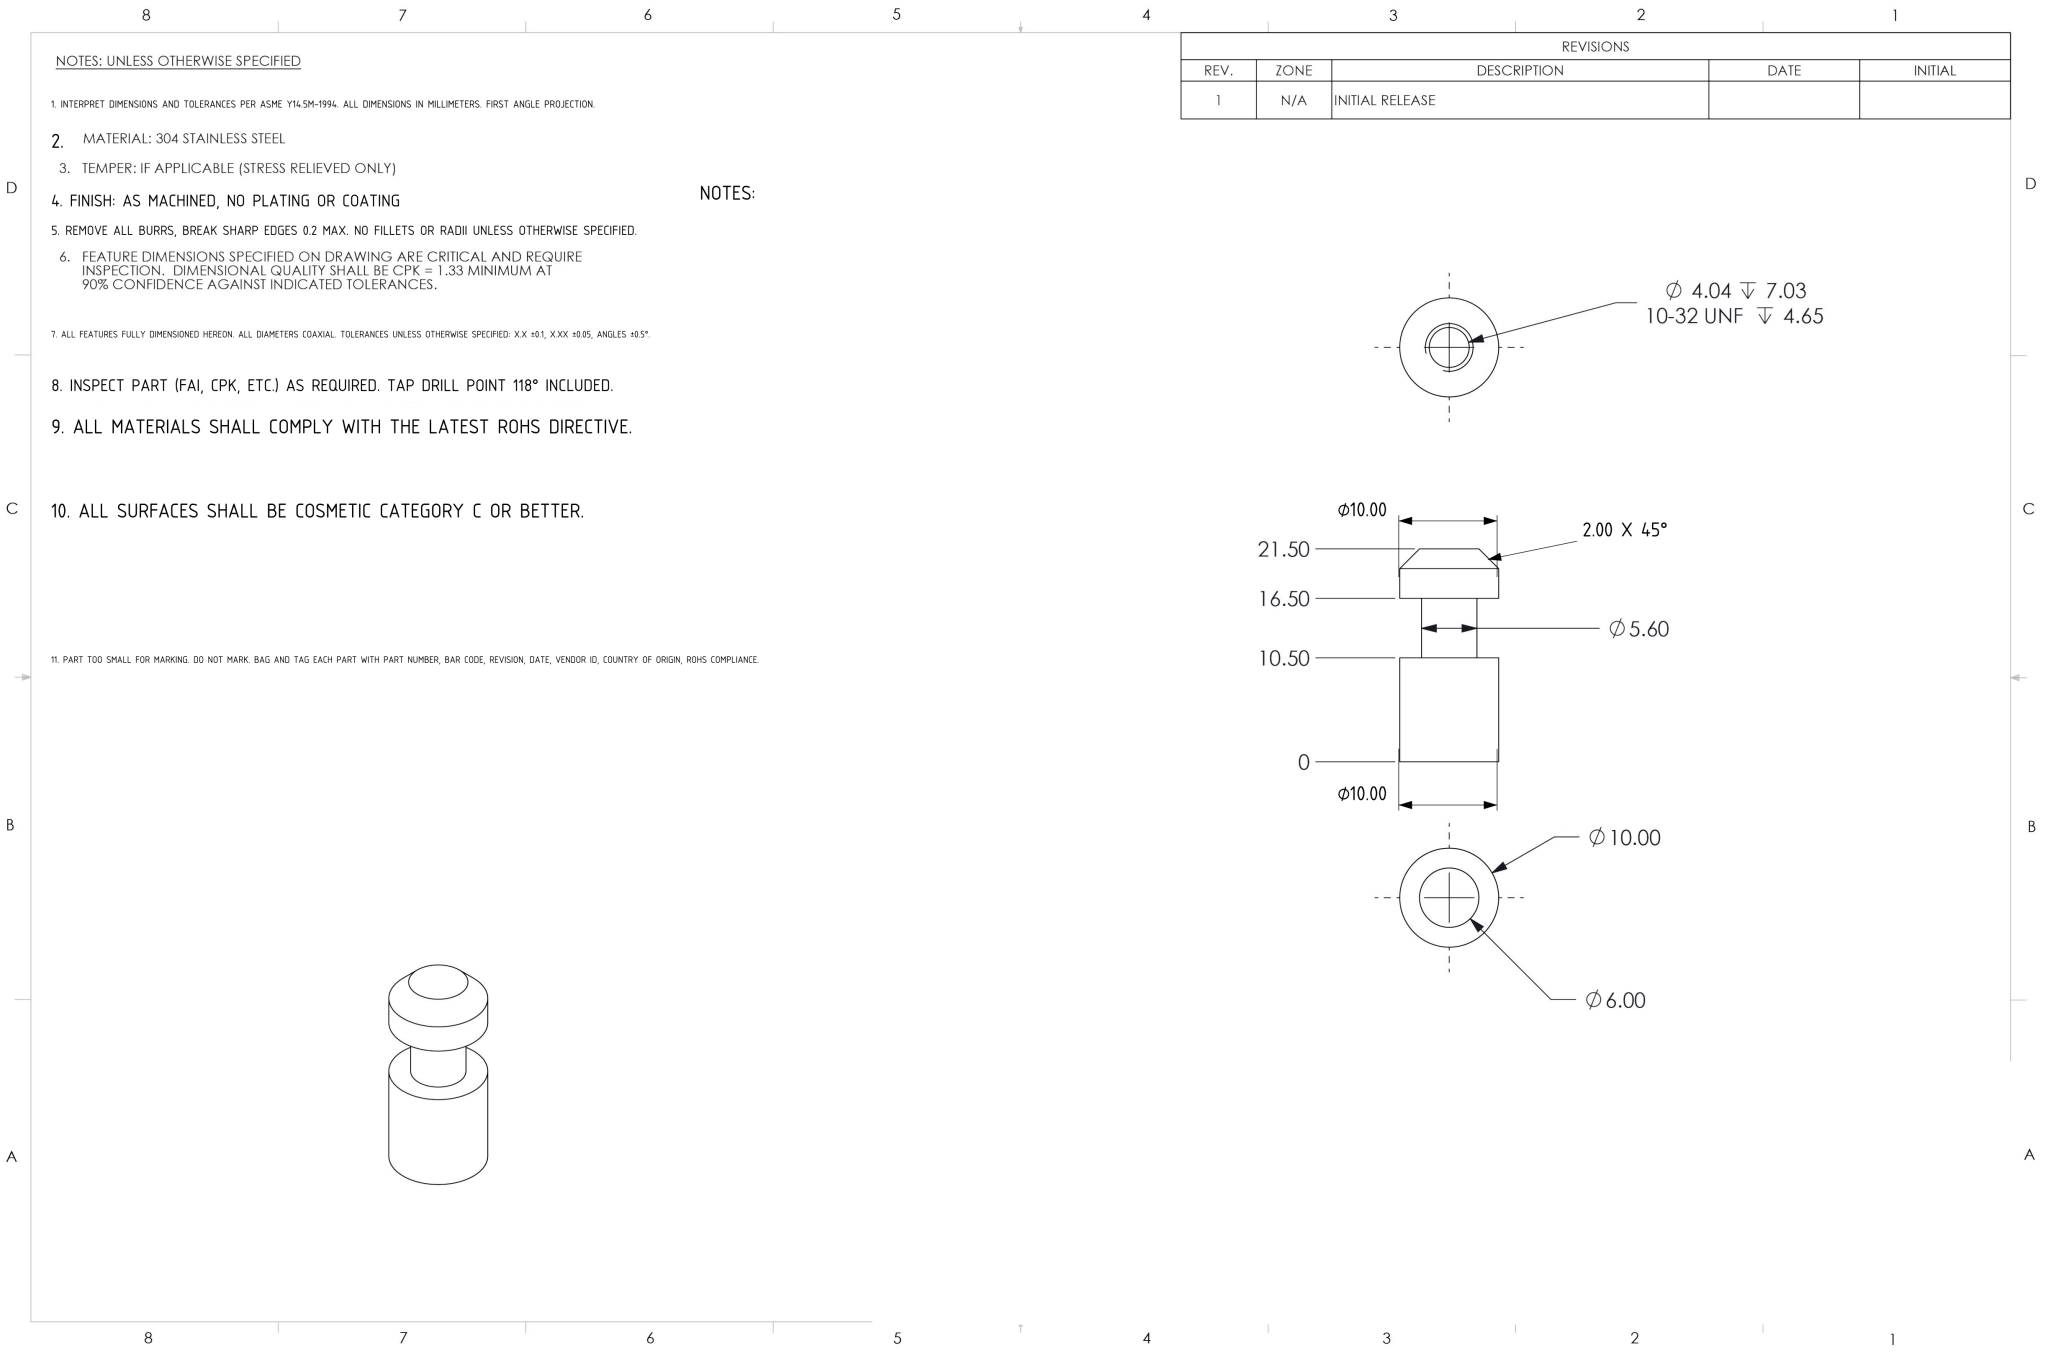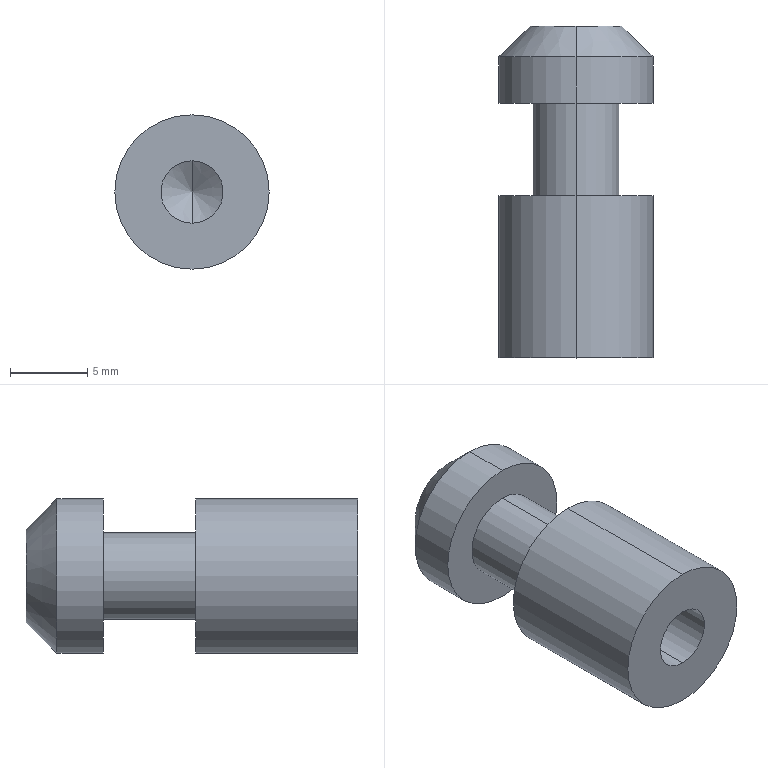Part | NX | drawing in metres | 1 solid | 16 faces | box 10 x 21.5 x 10 mm | volume 1215 mm3 | cylinder 8 | cone 4 | plane 4 | commonest cylinder face diameters 10 x4 4.039 x2 5.6 x2
STEP:
#1=COLOUR_RGB('',0.6471,0.6196,0.5843);
#2=FILL_AREA_STYLE_COLOUR('',#1);
#3=FILL_AREA_STYLE('',(#2));
#4=SURFACE_STYLE_FILL_AREA(#3);
#5=SURFACE_SIDE_STYLE('',(#4));
#6=SURFACE_STYLE_USAGE(.BOTH.,#5);
#7=PRESENTATION_STYLE_ASSIGNMENT((#6));
#8=CARTESIAN_POINT('',(0.,-0.01969,-0.1969));
#9=VERTEX_POINT('',#8);
#10=CARTESIAN_POINT('',(0.,-0.01969,0.1969));
#11=VERTEX_POINT('',#10);
#12=CARTESIAN_POINT('',(0.,-0.01969,0.));
#13=DIRECTION('',(0.,1.,0.));
#14=DIRECTION('',(0.,0.,-1.));
#15=AXIS2_PLACEMENT_3D('',#12,#13,#14);
#16=CIRCLE('',#15,0.1969);
#17=EDGE_CURVE('',#9,#11,#16,.T.);
#18=ORIENTED_EDGE('',*,*,#17,.F.);
#19=CARTESIAN_POINT('',(0.,-0.01969,0.));
#20=DIRECTION('',(0.,1.,0.));
#21=DIRECTION('',(0.,0.,-1.));
#22=AXIS2_PLACEMENT_3D('',#19,#20,#21);
#23=CIRCLE('',#22,0.1969);
#24=EDGE_CURVE('',#11,#9,#23,.T.);
#25=ORIENTED_EDGE('',*,*,#24,.F.);
#26=EDGE_LOOP('',(#18,#25));
#27=FACE_OUTER_BOUND('',#26,.T.);
#28=CARTESIAN_POINT('',(0.,-0.01969,-0.0795));
#29=VERTEX_POINT('',#28);
#30=CARTESIAN_POINT('',(0.,-0.01969,0.0795));
#31=VERTEX_POINT('',#30);
#32=CARTESIAN_POINT('',(0.,-0.01969,0.));
#33=DIRECTION('',(0.,1.,0.));
#34=DIRECTION('',(0.,0.,-1.));
#35=AXIS2_PLACEMENT_3D('',#32,#33,#34);
#36=CIRCLE('',#35,0.0795);
#37=EDGE_CURVE('',#29,#31,#36,.T.);
#38=ORIENTED_EDGE('',*,*,#37,.T.);
#39=CARTESIAN_POINT('',(0.,-0.01969,0.));
#40=DIRECTION('',(0.,1.,0.));
#41=DIRECTION('',(0.,0.,-1.));
#42=AXIS2_PLACEMENT_3D('',#39,#40,#41);
#43=CIRCLE('',#42,0.0795);
#44=EDGE_CURVE('',#31,#29,#43,.T.);
#45=ORIENTED_EDGE('',*,*,#44,.T.);
#46=EDGE_LOOP('',(#38,#45));
#47=FACE_BOUND('',#46,.T.);
#48=CARTESIAN_POINT('',(0.1969,-0.01969,0.));
#49=DIRECTION('',(0.,-1.,0.));
#50=DIRECTION('',(0.,0.,-1.));
#51=AXIS2_PLACEMENT_3D('',#48,#49,#50);
#52=PLANE('',#51);
#53=ADVANCED_FACE('',(#27,#47),#52,.T.);
#54=STYLED_ITEM('',(#7),#53);
#55=(LENGTH_UNIT()NAMED_UNIT(*)SI_UNIT($,.METRE.));
#56=LENGTH_MEASURE_WITH_UNIT(LENGTH_MEASURE(0.0254),#55);
#57=DIMENSIONAL_EXPONENTS(1.,0.,0.,0.,0.,0.,0.);
#58=(CONVERSION_BASED_UNIT('',#56)LENGTH_UNIT()NAMED_UNIT(#57));
#59=UNCERTAINTY_MEASURE_WITH_UNIT(LENGTH_MEASURE(0.00001),#58,'','');
#60=(NAMED_UNIT(*)PLANE_ANGLE_UNIT()SI_UNIT($,.RADIAN.));
#61=(NAMED_UNIT(*)SI_UNIT($,.STERADIAN.)SOLID_ANGLE_UNIT());
#62=(GEOMETRIC_REPRESENTATION_CONTEXT(3)GLOBAL_UNCERTAINTY_ASSIGNED_CONTEXT((#59))GLOBAL_UNIT_ASSIGNED_CONTEXT((#58,#60,#61))REPRESENTATION_CONTEXT('',''));
#63=MECHANICAL_DESIGN_GEOMETRIC_PRESENTATION_REPRESENTATION('',(#54),#62);
#64=COLOUR_RGB('',0.6471,0.6196,0.5843);
#65=FILL_AREA_STYLE_COLOUR('',#64);
#66=FILL_AREA_STYLE('',(#65));
#67=SURFACE_STYLE_FILL_AREA(#66);
#68=SURFACE_SIDE_STYLE('',(#67));
#69=SURFACE_STYLE_USAGE(.BOTH.,#68);
#70=PRESENTATION_STYLE_ASSIGNMENT((#69));
#71=CARTESIAN_POINT('',(0.,0.3049,0.));
#72=VERTEX_POINT('',#71);
#73=CARTESIAN_POINT('',(0.,0.2571,0.0795));
#74=VERTEX_POINT('',#73);
#75=CARTESIAN_POINT('',(0.,0.2571,0.0795));
#76=DIRECTION('',(0.,-0.515,0.8572));
#77=VECTOR('',#76,39.37);
#78=LINE('',#75,#77);
#79=EDGE_CURVE('',#72,#74,#78,.T.);
#80=ORIENTED_EDGE('',*,*,#79,.F.);
#81=CARTESIAN_POINT('',(0.,0.2571,-0.0795));
#82=VERTEX_POINT('',#81);
#83=CARTESIAN_POINT('',(0.,0.2571,-0.0795));
#84=DIRECTION('',(0.,-0.515,-0.8572));
#85=VECTOR('',#84,39.37);
#86=LINE('',#83,#85);
#87=EDGE_CURVE('',#72,#82,#86,.T.);
#88=ORIENTED_EDGE('',*,*,#87,.T.);
#89=CARTESIAN_POINT('',(0.,0.2571,0.));
#90=DIRECTION('',(0.,-1.,0.));
#91=DIRECTION('',(0.,0.,-1.));
#92=AXIS2_PLACEMENT_3D('',#89,#90,#91);
#93=CIRCLE('',#92,0.0795);
#94=EDGE_CURVE('',#82,#74,#93,.T.);
#95=ORIENTED_EDGE('',*,*,#94,.T.);
#96=EDGE_LOOP('',(#80,#88,#95));
#97=FACE_OUTER_BOUND('',#96,.T.);
#98=CARTESIAN_POINT('',(0.,0.2571,0.));
#99=DIRECTION('',(0.,-1.,0.));
#100=DIRECTION('',(0.,0.,-1.));
#101=AXIS2_PLACEMENT_3D('',#98,#99,#100);
#102=CONICAL_SURFACE('',#101,0.0795,1.03);
#103=ADVANCED_FACE('',(#97),#102,.F.);
#104=STYLED_ITEM('',(#70),#103);
#105=PRESENTATION_LAYER_ASSIGNMENT('','',(#104));
#106=COLOUR_RGB('',0.6471,0.6196,0.5843);
#107=FILL_AREA_STYLE_COLOUR('',#106);
#108=FILL_AREA_STYLE('',(#107));
#109=SURFACE_STYLE_FILL_AREA(#108);
#110=SURFACE_SIDE_STYLE('',(#109));
#111=SURFACE_STYLE_USAGE(.BOTH.,#110);
#112=PRESENTATION_STYLE_ASSIGNMENT((#111));
#113=CARTESIAN_POINT('',(0.,0.3937,-0.1969));
#114=VERTEX_POINT('',#113);
#115=CARTESIAN_POINT('',(0.,0.3937,0.1969));
#116=VERTEX_POINT('',#115);
#117=CARTESIAN_POINT('',(0.,0.3937,0.));
#118=DIRECTION('',(0.,-1.,0.));
#119=DIRECTION('',(0.,0.,-1.));
#120=AXIS2_PLACEMENT_3D('',#117,#118,#119);
#121=CIRCLE('',#120,0.1969);
#122=EDGE_CURVE('',#114,#116,#121,.T.);
#123=ORIENTED_EDGE('',*,*,#122,.T.);
#124=CARTESIAN_POINT('',(0.,0.,0.1969));
#125=DIRECTION('',(0.,-1.,0.));
#126=VECTOR('',#125,39.37);
#127=LINE('',#124,#126);
#128=EDGE_CURVE('',#116,#11,#127,.T.);
#129=ORIENTED_EDGE('',*,*,#128,.T.);
#130=ORIENTED_EDGE('',*,*,#24,.T.);
#131=CARTESIAN_POINT('',(0.,0.,-0.1969));
#132=DIRECTION('',(0.,-1.,0.));
#133=VECTOR('',#132,39.37);
#134=LINE('',#131,#133);
#135=EDGE_CURVE('',#114,#9,#134,.T.);
#136=ORIENTED_EDGE('',*,*,#135,.F.);
#137=EDGE_LOOP('',(#123,#129,#130,#136));
#138=FACE_OUTER_BOUND('',#137,.T.);
#139=CARTESIAN_POINT('',(0.,0.,0.));
#140=DIRECTION('',(0.,-1.,0.));
#141=DIRECTION('',(0.,0.,-1.));
#142=AXIS2_PLACEMENT_3D('',#139,#140,#141);
#143=CYLINDRICAL_SURFACE('',#142,0.1969);
#144=ADVANCED_FACE('',(#138),#143,.T.);
#145=STYLED_ITEM('',(#112),#144);
#146=(LENGTH_UNIT()NAMED_UNIT(*)SI_UNIT($,.METRE.));
#147=LENGTH_MEASURE_WITH_UNIT(LENGTH_MEASURE(0.0254),#146);
#148=DIMENSIONAL_EXPONENTS(1.,0.,0.,0.,0.,0.,0.);
#149=(CONVERSION_BASED_UNIT('',#147)LENGTH_UNIT()NAMED_UNIT(#148));
#150=UNCERTAINTY_MEASURE_WITH_UNIT(LENGTH_MEASURE(0.00001),#149,'','');
#151=(NAMED_UNIT(*)PLANE_ANGLE_UNIT()SI_UNIT($,.RADIAN.));
#152=(NAMED_UNIT(*)SI_UNIT($,.STERADIAN.)SOLID_ANGLE_UNIT());
#153=(GEOMETRIC_REPRESENTATION_CONTEXT(3)GLOBAL_UNCERTAINTY_ASSIGNED_CONTEXT((#150))GLOBAL_UNIT_ASSIGNED_CONTEXT((#149,#151,#152))REPRESENTATION_CONTEXT('',''));
#154=MECHANICAL_DESIGN_GEOMETRIC_PRESENTATION_REPRESENTATION('',(#145),#153);
#155=(LENGTH_UNIT()NAMED_UNIT(*)SI_UNIT($,.METRE.));
#156=LENGTH_MEASURE_WITH_UNIT(LENGTH_MEASURE(0.0254),#155);
#157=DIMENSIONAL_EXPONENTS(1.,0.,0.,0.,0.,0.,0.);
#158=(CONVERSION_BASED_UNIT('',#156)LENGTH_UNIT()NAMED_UNIT(#157));
#159=UNCERTAINTY_MEASURE_WITH_UNIT(LENGTH_MEASURE(0.00001),#158,'','');
#160=(NAMED_UNIT(*)PLANE_ANGLE_UNIT()SI_UNIT($,.RADIAN.));
#161=(NAMED_UNIT(*)SI_UNIT($,.STERADIAN.)SOLID_ANGLE_UNIT());
#162=(GEOMETRIC_REPRESENTATION_CONTEXT(3)GLOBAL_UNCERTAINTY_ASSIGNED_CONTEXT((#159))GLOBAL_UNIT_ASSIGNED_CONTEXT((#158,#160,#161))REPRESENTATION_CONTEXT('',''));
#163=MECHANICAL_DESIGN_GEOMETRIC_PRESENTATION_REPRESENTATION('',(#104),#162);
#164=COLOUR_RGB('',0.6471,0.6196,0.5843);
#165=FILL_AREA_STYLE_COLOUR('',#164);
#166=FILL_AREA_STYLE('',(#165));
#167=SURFACE_STYLE_FILL_AREA(#166);
#168=SURFACE_SIDE_STYLE('',(#167));
#169=SURFACE_STYLE_USAGE(.BOTH.,#168);
#170=PRESENTATION_STYLE_ASSIGNMENT((#169));
#171=CARTESIAN_POINT('',(0.,0.6299,-0.1102));
#172=VERTEX_POINT('',#171);
#173=CARTESIAN_POINT('',(0.,0.6299,0.1102));
#174=VERTEX_POINT('',#173);
#175=CARTESIAN_POINT('',(0.,0.6299,0.));
#176=DIRECTION('',(0.,-1.,0.));
#177=DIRECTION('',(0.,0.,-1.));
#178=AXIS2_PLACEMENT_3D('',#175,#176,#177);
#179=CIRCLE('',#178,0.1102);
#180=EDGE_CURVE('',#172,#174,#179,.T.);
#181=ORIENTED_EDGE('',*,*,#180,.T.);
#182=CARTESIAN_POINT('',(0.,0.3937,0.1102));
#183=VERTEX_POINT('',#182);
#184=CARTESIAN_POINT('',(0.,0.,0.1102));
#185=DIRECTION('',(0.,-1.,0.));
#186=VECTOR('',#185,39.37);
#187=LINE('',#184,#186);
#188=EDGE_CURVE('',#174,#183,#187,.T.);
#189=ORIENTED_EDGE('',*,*,#188,.T.);
#190=CARTESIAN_POINT('',(0.,0.3937,-0.1102));
#191=VERTEX_POINT('',#190);
#192=CARTESIAN_POINT('',(0.,0.3937,0.));
#193=DIRECTION('',(0.,-1.,0.));
#194=DIRECTION('',(0.,0.,-1.));
#195=AXIS2_PLACEMENT_3D('',#192,#193,#194);
#196=CIRCLE('',#195,0.1102);
#197=EDGE_CURVE('',#191,#183,#196,.T.);
#198=ORIENTED_EDGE('',*,*,#197,.F.);
#199=CARTESIAN_POINT('',(0.,0.,-0.1102));
#200=DIRECTION('',(0.,-1.,0.));
#201=VECTOR('',#200,39.37);
#202=LINE('',#199,#201);
#203=EDGE_CURVE('',#172,#191,#202,.T.);
#204=ORIENTED_EDGE('',*,*,#203,.F.);
#205=EDGE_LOOP('',(#181,#189,#198,#204));
#206=FACE_OUTER_BOUND('',#205,.T.);
#207=CARTESIAN_POINT('',(0.,0.,0.));
#208=DIRECTION('',(0.,-1.,0.));
#209=DIRECTION('',(0.,0.,-1.));
#210=AXIS2_PLACEMENT_3D('',#207,#208,#209);
#211=CYLINDRICAL_SURFACE('',#210,0.1102);
#212=ADVANCED_FACE('',(#206),#211,.T.);
#213=STYLED_ITEM('',(#170),#212);
#214=(LENGTH_UNIT()NAMED_UNIT(*)SI_UNIT($,.METRE.));
#215=LENGTH_MEASURE_WITH_UNIT(LENGTH_MEASURE(0.0254),#214);
#216=DIMENSIONAL_EXPONENTS(1.,0.,0.,0.,0.,0.,0.);
#217=(CONVERSION_BASED_UNIT('',#215)LENGTH_UNIT()NAMED_UNIT(#216));
#218=UNCERTAINTY_MEASURE_WITH_UNIT(LENGTH_MEASURE(0.00001),#217,'','');
#219=(NAMED_UNIT(*)PLANE_ANGLE_UNIT()SI_UNIT($,.RADIAN.));
#220=(NAMED_UNIT(*)SI_UNIT($,.STERADIAN.)SOLID_ANGLE_UNIT());
#221=(GEOMETRIC_REPRESENTATION_CONTEXT(3)GLOBAL_UNCERTAINTY_ASSIGNED_CONTEXT((#218))GLOBAL_UNIT_ASSIGNED_CONTEXT((#217,#219,#220))REPRESENTATION_CONTEXT('',''));
#222=MECHANICAL_DESIGN_GEOMETRIC_PRESENTATION_REPRESENTATION('',(#213),#221);
#223=COLOUR_RGB('',0.6471,0.6196,0.5843);
#224=FILL_AREA_STYLE_COLOUR('',#223);
#225=FILL_AREA_STYLE('',(#224));
#226=SURFACE_STYLE_FILL_AREA(#225);
#227=SURFACE_SIDE_STYLE('',(#226));
#228=SURFACE_STYLE_USAGE(.BOTH.,#227);
#229=PRESENTATION_STYLE_ASSIGNMENT((#228));
#230=CARTESIAN_POINT('',(0.,0.8268,-0.1181));
#231=VERTEX_POINT('',#230);
#232=CARTESIAN_POINT('',(0.,0.8268,0.1181));
#233=VERTEX_POINT('',#232);
#234=CARTESIAN_POINT('',(0.,0.8268,0.));
#235=DIRECTION('',(0.,-1.,0.));
#236=DIRECTION('',(0.,0.,-1.));
#237=AXIS2_PLACEMENT_3D('',#234,#235,#236);
#238=CIRCLE('',#237,0.1181);
#239=EDGE_CURVE('',#231,#233,#238,.T.);
#240=ORIENTED_EDGE('',*,*,#239,.F.);
#241=CARTESIAN_POINT('',(0.,0.8268,0.));
#242=DIRECTION('',(0.,-1.,0.));
#243=DIRECTION('',(0.,0.,-1.));
#244=AXIS2_PLACEMENT_3D('',#241,#242,#243);
#245=CIRCLE('',#244,0.1181);
#246=EDGE_CURVE('',#233,#231,#245,.T.);
#247=ORIENTED_EDGE('',*,*,#246,.F.);
#248=EDGE_LOOP('',(#240,#247));
#249=FACE_OUTER_BOUND('',#248,.T.);
#250=CARTESIAN_POINT('',(0.,0.8268,0.));
#251=DIRECTION('',(0.,1.,0.));
#252=DIRECTION('',(0.,0.,1.));
#253=AXIS2_PLACEMENT_3D('',#250,#251,#252);
#254=PLANE('',#253);
#255=ADVANCED_FACE('',(#249),#254,.T.);
#256=STYLED_ITEM('',(#229),#255);
#257=PRESENTATION_LAYER_ASSIGNMENT('','',(#256));
#258=COLOUR_RGB('',0.6471,0.6196,0.5843);
#259=FILL_AREA_STYLE_COLOUR('',#258);
#260=FILL_AREA_STYLE('',(#259));
#261=SURFACE_STYLE_FILL_AREA(#260);
#262=SURFACE_SIDE_STYLE('',(#261));
#263=SURFACE_STYLE_USAGE(.BOTH.,#262);
#264=PRESENTATION_STYLE_ASSIGNMENT((#263));
#265=ORIENTED_EDGE('',*,*,#239,.T.);
#266=CARTESIAN_POINT('',(0.,0.748,0.1969));
#267=VERTEX_POINT('',#266);
#268=CARTESIAN_POINT('',(0.,0.748,0.1969));
#269=DIRECTION('',(0.,-0.7071,0.7071));
#270=VECTOR('',#269,39.37);
#271=LINE('',#268,#270);
#272=EDGE_CURVE('',#233,#267,#271,.T.);
#273=ORIENTED_EDGE('',*,*,#272,.T.);
#274=CARTESIAN_POINT('',(0.,0.748,-0.1969));
#275=VERTEX_POINT('',#274);
#276=CARTESIAN_POINT('',(0.,0.748,0.));
#277=DIRECTION('',(0.,-1.,0.));
#278=DIRECTION('',(0.,0.,-1.));
#279=AXIS2_PLACEMENT_3D('',#276,#277,#278);
#280=CIRCLE('',#279,0.1969);
#281=EDGE_CURVE('',#275,#267,#280,.T.);
#282=ORIENTED_EDGE('',*,*,#281,.F.);
#283=CARTESIAN_POINT('',(0.,0.748,-0.1969));
#284=DIRECTION('',(0.,-0.7071,-0.7071));
#285=VECTOR('',#284,39.37);
#286=LINE('',#283,#285);
#287=EDGE_CURVE('',#231,#275,#286,.T.);
#288=ORIENTED_EDGE('',*,*,#287,.F.);
#289=EDGE_LOOP('',(#265,#273,#282,#288));
#290=FACE_OUTER_BOUND('',#289,.T.);
#291=CARTESIAN_POINT('',(0.,0.748,0.));
#292=DIRECTION('',(0.,-1.,0.));
#293=DIRECTION('',(0.,0.,-1.));
#294=AXIS2_PLACEMENT_3D('',#291,#292,#293);
#295=CONICAL_SURFACE('',#294,0.1969,0.7854);
#296=ADVANCED_FACE('',(#290),#295,.T.);
#297=STYLED_ITEM('',(#264),#296);
#298=PRESENTATION_LAYER_ASSIGNMENT('','',(#297));
#299=COLOUR_RGB('',0.6471,0.6196,0.5843);
#300=FILL_AREA_STYLE_COLOUR('',#299);
#301=FILL_AREA_STYLE('',(#300));
#302=SURFACE_STYLE_FILL_AREA(#301);
#303=SURFACE_SIDE_STYLE('',(#302));
#304=SURFACE_STYLE_USAGE(.BOTH.,#303);
#305=PRESENTATION_STYLE_ASSIGNMENT((#304));
#306=ORIENTED_EDGE('',*,*,#180,.F.);
#307=CARTESIAN_POINT('',(0.,0.6299,0.));
#308=DIRECTION('',(0.,-1.,0.));
#309=DIRECTION('',(0.,0.,-1.));
#310=AXIS2_PLACEMENT_3D('',#307,#308,#309);
#311=CIRCLE('',#310,0.1102);
#312=EDGE_CURVE('',#174,#172,#311,.T.);
#313=ORIENTED_EDGE('',*,*,#312,.F.);
#314=EDGE_LOOP('',(#306,#313));
#315=FACE_BOUND('',#314,.T.);
#316=CARTESIAN_POINT('',(0.,0.6299,-0.1969));
#317=VERTEX_POINT('',#316);
#318=CARTESIAN_POINT('',(0.,0.6299,0.1969));
#319=VERTEX_POINT('',#318);
#320=CARTESIAN_POINT('',(0.,0.6299,0.));
#321=DIRECTION('',(0.,-1.,0.));
#322=DIRECTION('',(0.,0.,-1.));
#323=AXIS2_PLACEMENT_3D('',#320,#321,#322);
#324=CIRCLE('',#323,0.1969);
#325=EDGE_CURVE('',#317,#319,#324,.T.);
#326=ORIENTED_EDGE('',*,*,#325,.T.);
#327=CARTESIAN_POINT('',(0.,0.6299,0.));
#328=DIRECTION('',(0.,-1.,0.));
#329=DIRECTION('',(0.,0.,-1.));
#330=AXIS2_PLACEMENT_3D('',#327,#328,#329);
#331=CIRCLE('',#330,0.1969);
#332=EDGE_CURVE('',#319,#317,#331,.T.);
#333=ORIENTED_EDGE('',*,*,#332,.T.);
#334=EDGE_LOOP('',(#326,#333));
#335=FACE_OUTER_BOUND('',#334,.T.);
#336=CARTESIAN_POINT('',(0.1969,0.6299,0.));
#337=DIRECTION('',(0.,-1.,0.));
#338=DIRECTION('',(0.,0.,-1.));
#339=AXIS2_PLACEMENT_3D('',#336,#337,#338);
#340=PLANE('',#339);
#341=ADVANCED_FACE('',(#315,#335),#340,.T.);
#342=STYLED_ITEM('',(#305),#341);
#343=PRESENTATION_LAYER_ASSIGNMENT('','',(#342));
#344=(LENGTH_UNIT()NAMED_UNIT(*)SI_UNIT($,.METRE.));
#345=LENGTH_MEASURE_WITH_UNIT(LENGTH_MEASURE(0.0254),#344);
#346=DIMENSIONAL_EXPONENTS(1.,0.,0.,0.,0.,0.,0.);
#347=(CONVERSION_BASED_UNIT('',#345)LENGTH_UNIT()NAMED_UNIT(#346));
#348=UNCERTAINTY_MEASURE_WITH_UNIT(LENGTH_MEASURE(0.00001),#347,'','');
#349=(NAMED_UNIT(*)PLANE_ANGLE_UNIT()SI_UNIT($,.RADIAN.));
#350=(NAMED_UNIT(*)SI_UNIT($,.STERADIAN.)SOLID_ANGLE_UNIT());
#351=(GEOMETRIC_REPRESENTATION_CONTEXT(3)GLOBAL_UNCERTAINTY_ASSIGNED_CONTEXT((#348))GLOBAL_UNIT_ASSIGNED_CONTEXT((#347,#349,#350))REPRESENTATION_CONTEXT('',''));
#352=MECHANICAL_DESIGN_GEOMETRIC_PRESENTATION_REPRESENTATION('',(#256),#351);
#353=(LENGTH_UNIT()NAMED_UNIT(*)SI_UNIT($,.METRE.));
#354=LENGTH_MEASURE_WITH_UNIT(LENGTH_MEASURE(0.0254),#353);
#355=DIMENSIONAL_EXPONENTS(1.,0.,0.,0.,0.,0.,0.);
#356=(CONVERSION_BASED_UNIT('',#354)LENGTH_UNIT()NAMED_UNIT(#355));
#357=UNCERTAINTY_MEASURE_WITH_UNIT(LENGTH_MEASURE(0.00001),#356,'','');
#358=(NAMED_UNIT(*)PLANE_ANGLE_UNIT()SI_UNIT($,.RADIAN.));
#359=(NAMED_UNIT(*)SI_UNIT($,.STERADIAN.)SOLID_ANGLE_UNIT());
#360=(GEOMETRIC_REPRESENTATION_CONTEXT(3)GLOBAL_UNCERTAINTY_ASSIGNED_CONTEXT((#357))GLOBAL_UNIT_ASSIGNED_CONTEXT((#356,#358,#359))REPRESENTATION_CONTEXT('',''));
#361=MECHANICAL_DESIGN_GEOMETRIC_PRESENTATION_REPRESENTATION('',(#297),#360);
#362=(LENGTH_UNIT()NAMED_UNIT(*)SI_UNIT($,.METRE.));
#363=LENGTH_MEASURE_WITH_UNIT(LENGTH_MEASURE(0.0254),#362);
#364=DIMENSIONAL_EXPONENTS(1.,0.,0.,0.,0.,0.,0.);
#365=(CONVERSION_BASED_UNIT('',#363)LENGTH_UNIT()NAMED_UNIT(#364));
#366=UNCERTAINTY_MEASURE_WITH_UNIT(LENGTH_MEASURE(0.00001),#365,'','');
#367=(NAMED_UNIT(*)PLANE_ANGLE_UNIT()SI_UNIT($,.RADIAN.));
#368=(NAMED_UNIT(*)SI_UNIT($,.STERADIAN.)SOLID_ANGLE_UNIT());
#369=(GEOMETRIC_REPRESENTATION_CONTEXT(3)GLOBAL_UNCERTAINTY_ASSIGNED_CONTEXT((#366))GLOBAL_UNIT_ASSIGNED_CONTEXT((#365,#367,#368))REPRESENTATION_CONTEXT('',''));
#370=MECHANICAL_DESIGN_GEOMETRIC_PRESENTATION_REPRESENTATION('',(#342),#369);
#371=COLOUR_RGB('',0.6471,0.6196,0.5843);
#372=FILL_AREA_STYLE_COLOUR('',#371);
#373=FILL_AREA_STYLE('',(#372));
#374=SURFACE_STYLE_FILL_AREA(#373);
#375=SURFACE_SIDE_STYLE('',(#374));
#376=SURFACE_STYLE_USAGE(.BOTH.,#375);
#377=PRESENTATION_STYLE_ASSIGNMENT((#376));
#378=ORIENTED_EDGE('',*,*,#281,.T.);
#379=CARTESIAN_POINT('',(0.,0.,0.1969));
#380=DIRECTION('',(0.,-1.,0.));
#381=VECTOR('',#380,39.37);
#382=LINE('',#379,#381);
#383=EDGE_CURVE('',#267,#319,#382,.T.);
#384=ORIENTED_EDGE('',*,*,#383,.T.);
#385=ORIENTED_EDGE('',*,*,#325,.F.);
#386=CARTESIAN_POINT('',(0.,0.,-0.1969));
#387=DIRECTION('',(0.,-1.,0.));
#388=VECTOR('',#387,39.37);
#389=LINE('',#386,#388);
#390=EDGE_CURVE('',#275,#317,#389,.T.);
#391=ORIENTED_EDGE('',*,*,#390,.F.);
#392=EDGE_LOOP('',(#378,#384,#385,#391));
#393=FACE_OUTER_BOUND('',#392,.T.);
#394=CARTESIAN_POINT('',(0.,0.,0.));
#395=DIRECTION('',(0.,-1.,0.));
#396=DIRECTION('',(0.,0.,-1.));
#397=AXIS2_PLACEMENT_3D('',#394,#395,#396);
#398=CYLINDRICAL_SURFACE('',#397,0.1969);
#399=ADVANCED_FACE('',(#393),#398,.T.);
#400=STYLED_ITEM('',(#377),#399);
#401=PRESENTATION_LAYER_ASSIGNMENT('','',(#400));
#402=(LENGTH_UNIT()NAMED_UNIT(*)SI_UNIT($,.METRE.));
#403=LENGTH_MEASURE_WITH_UNIT(LENGTH_MEASURE(0.0254),#402);
#404=DIMENSIONAL_EXPONENTS(1.,0.,0.,0.,0.,0.,0.);
#405=(CONVERSION_BASED_UNIT('',#403)LENGTH_UNIT()NAMED_UNIT(#404));
#406=UNCERTAINTY_MEASURE_WITH_UNIT(LENGTH_MEASURE(0.00001),#405,'','');
#407=(NAMED_UNIT(*)PLANE_ANGLE_UNIT()SI_UNIT($,.RADIAN.));
#408=(NAMED_UNIT(*)SI_UNIT($,.STERADIAN.)SOLID_ANGLE_UNIT());
#409=(GEOMETRIC_REPRESENTATION_CONTEXT(3)GLOBAL_UNCERTAINTY_ASSIGNED_CONTEXT((#406))GLOBAL_UNIT_ASSIGNED_CONTEXT((#405,#407,#408))REPRESENTATION_CONTEXT('',''));
#410=MECHANICAL_DESIGN_GEOMETRIC_PRESENTATION_REPRESENTATION('',(#400),#409);
#411=COLOUR_RGB('',0.6471,0.6196,0.5843);
#412=FILL_AREA_STYLE_COLOUR('',#411);
#413=FILL_AREA_STYLE('',(#412));
#414=SURFACE_STYLE_FILL_AREA(#413);
#415=SURFACE_SIDE_STYLE('',(#414));
#416=SURFACE_STYLE_USAGE(.BOTH.,#415);
#417=PRESENTATION_STYLE_ASSIGNMENT((#416));
#418=ORIENTED_EDGE('',*,*,#128,.F.);
#419=CARTESIAN_POINT('',(0.,0.3937,0.));
#420=DIRECTION('',(0.,-1.,0.));
#421=DIRECTION('',(0.,0.,-1.));
#422=AXIS2_PLACEMENT_3D('',#419,#420,#421);
#423=CIRCLE('',#422,0.1969);
#424=EDGE_CURVE('',#116,#114,#423,.T.);
#425=ORIENTED_EDGE('',*,*,#424,.T.);
#426=ORIENTED_EDGE('',*,*,#135,.T.);
#427=ORIENTED_EDGE('',*,*,#17,.T.);
#428=EDGE_LOOP('',(#418,#425,#426,#427));
#429=FACE_OUTER_BOUND('',#428,.T.);
#430=CARTESIAN_POINT('',(0.,0.,0.));
#431=DIRECTION('',(0.,-1.,0.));
#432=DIRECTION('',(0.,0.,-1.));
#433=AXIS2_PLACEMENT_3D('',#430,#431,#432);
#434=CYLINDRICAL_SURFACE('',#433,0.1969);
#435=ADVANCED_FACE('',(#429),#434,.T.);
#436=STYLED_ITEM('',(#417),#435);
#437=PRESENTATION_LAYER_ASSIGNMENT('','',(#436));
#438=COLOUR_RGB('',0.6471,0.6196,0.5843);
#439=FILL_AREA_STYLE_COLOUR('',#438);
#440=FILL_AREA_STYLE('',(#439));
#441=SURFACE_STYLE_FILL_AREA(#440);
#442=SURFACE_SIDE_STYLE('',(#441));
#443=SURFACE_STYLE_USAGE(.BOTH.,#442);
#444=PRESENTATION_STYLE_ASSIGNMENT((#443));
#445=CARTESIAN_POINT('',(0.,0.2571,0.));
#446=DIRECTION('',(0.,-1.,0.));
#447=DIRECTION('',(0.,0.,-1.));
#448=AXIS2_PLACEMENT_3D('',#445,#446,#447);
#449=CIRCLE('',#448,0.0795);
#450=EDGE_CURVE('',#74,#82,#449,.T.);
#451=ORIENTED_EDGE('',*,*,#450,.F.);
#452=CARTESIAN_POINT('',(0.,-0.01969,0.0795));
#453=DIRECTION('',(0.,-1.,0.));
#454=VECTOR('',#453,39.37);
#455=LINE('',#452,#454);
#456=EDGE_CURVE('',#74,#31,#455,.T.);
#457=ORIENTED_EDGE('',*,*,#456,.T.);
#458=ORIENTED_EDGE('',*,*,#37,.F.);
#459=CARTESIAN_POINT('',(0.,-0.01969,-0.0795));
#460=DIRECTION('',(0.,-1.,0.));
#461=VECTOR('',#460,39.37);
#462=LINE('',#459,#461);
#463=EDGE_CURVE('',#82,#29,#462,.T.);
#464=ORIENTED_EDGE('',*,*,#463,.F.);
#465=EDGE_LOOP('',(#451,#457,#458,#464));
#466=FACE_OUTER_BOUND('',#465,.T.);
#467=CARTESIAN_POINT('',(0.,-0.01969,0.));
#468=DIRECTION('',(0.,-1.,0.));
#469=DIRECTION('',(0.,0.,-1.));
#470=AXIS2_PLACEMENT_3D('',#467,#468,#469);
#471=CYLINDRICAL_SURFACE('',#470,0.0795);
#472=ADVANCED_FACE('',(#466),#471,.F.);
#473=STYLED_ITEM('',(#444),#472);
#474=PRESENTATION_LAYER_ASSIGNMENT('','',(#473));
#475=(LENGTH_UNIT()NAMED_UNIT(*)SI_UNIT($,.METRE.));
#476=LENGTH_MEASURE_WITH_UNIT(LENGTH_MEASURE(0.0254),#475);
#477=DIMENSIONAL_EXPONENTS(1.,0.,0.,0.,0.,0.,0.);
#478=(CONVERSION_BASED_UNIT('',#476)LENGTH_UNIT()NAMED_UNIT(#477));
#479=UNCERTAINTY_MEASURE_WITH_UNIT(LENGTH_MEASURE(0.00001),#478,'','');
#480=(NAMED_UNIT(*)PLANE_ANGLE_UNIT()SI_UNIT($,.RADIAN.));
#481=(NAMED_UNIT(*)SI_UNIT($,.STERADIAN.)SOLID_ANGLE_UNIT());
#482=(GEOMETRIC_REPRESENTATION_CONTEXT(3)GLOBAL_UNCERTAINTY_ASSIGNED_CONTEXT((#479))GLOBAL_UNIT_ASSIGNED_CONTEXT((#478,#480,#481))REPRESENTATION_CONTEXT('',''));
#483=MECHANICAL_DESIGN_GEOMETRIC_PRESENTATION_REPRESENTATION('',(#436),#482);
#484=COLOUR_RGB('',0.6471,0.6196,0.5843);
#485=FILL_AREA_STYLE_COLOUR('',#484);
#486=FILL_AREA_STYLE('',(#485));
#487=SURFACE_STYLE_FILL_AREA(#486);
#488=SURFACE_SIDE_STYLE('',(#487));
#489=SURFACE_STYLE_USAGE(.BOTH.,#488);
#490=PRESENTATION_STYLE_ASSIGNMENT((#489));
#491=ORIENTED_EDGE('',*,*,#456,.F.);
#492=ORIENTED_EDGE('',*,*,#94,.F.);
#493=ORIENTED_EDGE('',*,*,#463,.T.);
#494=ORIENTED_EDGE('',*,*,#44,.F.);
#495=EDGE_LOOP('',(#491,#492,#493,#494));
#496=FACE_OUTER_BOUND('',#495,.T.);
#497=CARTESIAN_POINT('',(0.,-0.01969,0.));
#498=DIRECTION('',(0.,-1.,0.));
#499=DIRECTION('',(0.,0.,-1.));
#500=AXIS2_PLACEMENT_3D('',#497,#498,#499);
#501=CYLINDRICAL_SURFACE('',#500,0.0795);
#502=ADVANCED_FACE('',(#496),#501,.F.);
#503=STYLED_ITEM('',(#490),#502);
#504=PRESENTATION_LAYER_ASSIGNMENT('','',(#503));
#505=COLOUR_RGB('',0.6471,0.6196,0.5843);
#506=FILL_AREA_STYLE_COLOUR('',#505);
#507=FILL_AREA_STYLE('',(#506));
#508=SURFACE_STYLE_FILL_AREA(#507);
#509=SURFACE_SIDE_STYLE('',(#508));
#510=SURFACE_STYLE_USAGE(.BOTH.,#509);
#511=PRESENTATION_STYLE_ASSIGNMENT((#510));
#512=ORIENTED_EDGE('',*,*,#122,.F.);
#513=ORIENTED_EDGE('',*,*,#424,.F.);
#514=EDGE_LOOP('',(#512,#513));
#515=FACE_OUTER_BOUND('',#514,.T.);
#516=ORIENTED_EDGE('',*,*,#197,.T.);
#517=CARTESIAN_POINT('',(0.,0.3937,0.));
#518=DIRECTION('',(0.,-1.,0.));
#519=DIRECTION('',(0.,0.,-1.));
#520=AXIS2_PLACEMENT_3D('',#517,#518,#519);
#521=CIRCLE('',#520,0.1102);
#522=EDGE_CURVE('',#183,#191,#521,.T.);
#523=ORIENTED_EDGE('',*,*,#522,.T.);
#524=EDGE_LOOP('',(#516,#523));
#525=FACE_BOUND('',#524,.T.);
#526=CARTESIAN_POINT('',(0.1102,0.3937,0.));
#527=DIRECTION('',(0.,1.,0.));
#528=DIRECTION('',(0.,0.,1.));
#529=AXIS2_PLACEMENT_3D('',#526,#527,#528);
#530=PLANE('',#529);
#531=ADVANCED_FACE('',(#515,#525),#530,.T.);
#532=STYLED_ITEM('',(#511),#531);
#533=PRESENTATION_LAYER_ASSIGNMENT('','',(#532));
#534=(LENGTH_UNIT()NAMED_UNIT(*)SI_UNIT($,.METRE.));
#535=LENGTH_MEASURE_WITH_UNIT(LENGTH_MEASURE(0.0254),#534);
#536=DIMENSIONAL_EXPONENTS(1.,0.,0.,0.,0.,0.,0.);
#537=(CONVERSION_BASED_UNIT('',#535)LENGTH_UNIT()NAMED_UNIT(#536));
#538=UNCERTAINTY_MEASURE_WITH_UNIT(LENGTH_MEASURE(0.00001),#537,'','');
#539=(NAMED_UNIT(*)PLANE_ANGLE_UNIT()SI_UNIT($,.RADIAN.));
#540=(NAMED_UNIT(*)SI_UNIT($,.STERADIAN.)SOLID_ANGLE_UNIT());
#541=(GEOMETRIC_REPRESENTATION_CONTEXT(3)GLOBAL_UNCERTAINTY_ASSIGNED_CONTEXT((#538))GLOBAL_UNIT_ASSIGNED_CONTEXT((#537,#539,#540))REPRESENTATION_CONTEXT('',''));
#542=MECHANICAL_DESIGN_GEOMETRIC_PRESENTATION_REPRESENTATION('',(#473),#541);
#543=(LENGTH_UNIT()NAMED_UNIT(*)SI_UNIT($,.METRE.));
#544=LENGTH_MEASURE_WITH_UNIT(LENGTH_MEASURE(0.0254),#543);
#545=DIMENSIONAL_EXPONENTS(1.,0.,0.,0.,0.,0.,0.);
#546=(CONVERSION_BASED_UNIT('',#544)LENGTH_UNIT()NAMED_UNIT(#545));
#547=UNCERTAINTY_MEASURE_WITH_UNIT(LENGTH_MEASURE(0.00001),#546,'','');
#548=(NAMED_UNIT(*)PLANE_ANGLE_UNIT()SI_UNIT($,.RADIAN.));
#549=(NAMED_UNIT(*)SI_UNIT($,.STERADIAN.)SOLID_ANGLE_UNIT());
#550=(GEOMETRIC_REPRESENTATION_CONTEXT(3)GLOBAL_UNCERTAINTY_ASSIGNED_CONTEXT((#547))GLOBAL_UNIT_ASSIGNED_CONTEXT((#546,#548,#549))REPRESENTATION_CONTEXT('',''));
#551=MECHANICAL_DESIGN_GEOMETRIC_PRESENTATION_REPRESENTATION('',(#532),#550);
#552=COLOUR_RGB('',0.7922,0.8196,0.9333);
#553=FILL_AREA_STYLE_COLOUR('',#552);
#554=FILL_AREA_STYLE('',(#553));
#555=SURFACE_STYLE_FILL_AREA(#554);
#556=SURFACE_SIDE_STYLE('',(#555));
#557=SURFACE_STYLE_USAGE(.BOTH.,#556);
#558=PRESENTATION_STYLE_ASSIGNMENT((#557));
#559=ORIENTED_EDGE('',*,*,#87,.F.);
#560=ORIENTED_EDGE('',*,*,#79,.T.);
#561=ORIENTED_EDGE('',*,*,#450,.T.);
#562=EDGE_LOOP('',(#559,#560,#561));
#563=FACE_OUTER_BOUND('',#562,.T.);
#564=CARTESIAN_POINT('',(0.,0.2571,0.));
#565=DIRECTION('',(0.,-1.,0.));
#566=DIRECTION('',(0.,0.,-1.));
#567=AXIS2_PLACEMENT_3D('',#564,#565,#566);
#568=CONICAL_SURFACE('',#567,0.0795,1.03);
#569=ADVANCED_FACE('',(#563),#568,.F.);
#570=ORIENTED_EDGE('',*,*,#188,.F.);
#571=ORIENTED_EDGE('',*,*,#312,.T.);
#572=ORIENTED_EDGE('',*,*,#203,.T.);
#573=ORIENTED_EDGE('',*,*,#522,.F.);
#574=EDGE_LOOP('',(#570,#571,#572,#573));
#575=FACE_OUTER_BOUND('',#574,.T.);
#576=CARTESIAN_POINT('',(0.,0.,0.));
#577=DIRECTION('',(0.,-1.,0.));
#578=DIRECTION('',(0.,0.,-1.));
#579=AXIS2_PLACEMENT_3D('',#576,#577,#578);
#580=CYLINDRICAL_SURFACE('',#579,0.1102);
#581=ADVANCED_FACE('',(#575),#580,.T.);
#582=ORIENTED_EDGE('',*,*,#383,.F.);
#583=CARTESIAN_POINT('',(0.,0.748,0.));
#584=DIRECTION('',(0.,-1.,0.));
#585=DIRECTION('',(0.,0.,-1.));
#586=AXIS2_PLACEMENT_3D('',#583,#584,#585);
#587=CIRCLE('',#586,0.1969);
#588=EDGE_CURVE('',#267,#275,#587,.T.);
#589=ORIENTED_EDGE('',*,*,#588,.T.);
#590=ORIENTED_EDGE('',*,*,#390,.T.);
#591=ORIENTED_EDGE('',*,*,#332,.F.);
#592=EDGE_LOOP('',(#582,#589,#590,#591));
#593=FACE_OUTER_BOUND('',#592,.T.);
#594=CARTESIAN_POINT('',(0.,0.,0.));
#595=DIRECTION('',(0.,-1.,0.));
#596=DIRECTION('',(0.,0.,-1.));
#597=AXIS2_PLACEMENT_3D('',#594,#595,#596);
#598=CYLINDRICAL_SURFACE('',#597,0.1969);
#599=ADVANCED_FACE('',(#593),#598,.T.);
#600=ORIENTED_EDGE('',*,*,#272,.F.);
#601=ORIENTED_EDGE('',*,*,#246,.T.);
#602=ORIENTED_EDGE('',*,*,#287,.T.);
#603=ORIENTED_EDGE('',*,*,#588,.F.);
#604=EDGE_LOOP('',(#600,#601,#602,#603));
#605=FACE_OUTER_BOUND('',#604,.T.);
#606=CARTESIAN_POINT('',(0.,0.748,0.));
#607=DIRECTION('',(0.,-1.,0.));
#608=DIRECTION('',(0.,0.,-1.));
#609=AXIS2_PLACEMENT_3D('',#606,#607,#608);
#610=CONICAL_SURFACE('',#609,0.1969,0.7854);
#611=ADVANCED_FACE('',(#605),#610,.T.);
#612=CLOSED_SHELL('',(#144,#472,#212,#569,#399,#296,#435,#53,#531,#502,#581,#103,#341,#599,#611,#255));
#613=MANIFOLD_SOLID_BREP('',#612);
#614=CARTESIAN_POINT('',(0.,0.,0.));
#615=DIRECTION('',(0.,0.,1.));
#616=DIRECTION('',(1.,0.,0.));
#617=AXIS2_PLACEMENT_3D('',#614,#615,#616);
#618=(LENGTH_UNIT()NAMED_UNIT(*)SI_UNIT($,.METRE.));
#619=LENGTH_MEASURE_WITH_UNIT(LENGTH_MEASURE(0.0254),#618);
#620=DIMENSIONAL_EXPONENTS(1.,0.,0.,0.,0.,0.,0.);
#621=(CONVERSION_BASED_UNIT('',#619)LENGTH_UNIT()NAMED_UNIT(#620));
#622=UNCERTAINTY_MEASURE_WITH_UNIT(LENGTH_MEASURE(0.00001),#621,'','');
#623=(NAMED_UNIT(*)PLANE_ANGLE_UNIT()SI_UNIT($,.RADIAN.));
#624=(NAMED_UNIT(*)SI_UNIT($,.STERADIAN.)SOLID_ANGLE_UNIT());
#625=(GEOMETRIC_REPRESENTATION_CONTEXT(3)GLOBAL_UNCERTAINTY_ASSIGNED_CONTEXT((#622))GLOBAL_UNIT_ASSIGNED_CONTEXT((#621,#623,#624))REPRESENTATION_CONTEXT('',''));
#626=ADVANCED_BREP_SHAPE_REPRESENTATION('',(#613,#617),#625);
#627=STYLED_ITEM('',(#558),#626);
#628=PRESENTATION_LAYER_ASSIGNMENT('','',(#627));
#629=COLOUR_RGB('',0.6471,0.6196,0.5843);
#630=FILL_AREA_STYLE_COLOUR('',#629);
#631=FILL_AREA_STYLE('',(#630));
#632=SURFACE_STYLE_FILL_AREA(#631);
#633=SURFACE_SIDE_STYLE('',(#632));
#634=SURFACE_STYLE_USAGE(.BOTH.,#633);
#635=PRESENTATION_STYLE_ASSIGNMENT((#634));
#636=STYLED_ITEM('',(#635),#569);
#637=PRESENTATION_LAYER_ASSIGNMENT('','',(#636));
#638=COLOUR_RGB('',0.6471,0.6196,0.5843);
#639=FILL_AREA_STYLE_COLOUR('',#638);
#640=FILL_AREA_STYLE('',(#639));
#641=SURFACE_STYLE_FILL_AREA(#640);
#642=SURFACE_SIDE_STYLE('',(#641));
#643=SURFACE_STYLE_USAGE(.BOTH.,#642);
#644=PRESENTATION_STYLE_ASSIGNMENT((#643));
#645=STYLED_ITEM('',(#644),#581);
#646=PRESENTATION_LAYER_ASSIGNMENT('','',(#645));
#647=(LENGTH_UNIT()NAMED_UNIT(*)SI_UNIT($,.METRE.));
#648=LENGTH_MEASURE_WITH_UNIT(LENGTH_MEASURE(0.0254),#647);
#649=DIMENSIONAL_EXPONENTS(1.,0.,0.,0.,0.,0.,0.);
#650=(CONVERSION_BASED_UNIT('',#648)LENGTH_UNIT()NAMED_UNIT(#649));
#651=UNCERTAINTY_MEASURE_WITH_UNIT(LENGTH_MEASURE(0.00001),#650,'','');
#652=(NAMED_UNIT(*)PLANE_ANGLE_UNIT()SI_UNIT($,.RADIAN.));
#653=(NAMED_UNIT(*)SI_UNIT($,.STERADIAN.)SOLID_ANGLE_UNIT());
#654=(GEOMETRIC_REPRESENTATION_CONTEXT(3)GLOBAL_UNCERTAINTY_ASSIGNED_CONTEXT((#651))GLOBAL_UNIT_ASSIGNED_CONTEXT((#650,#652,#653))REPRESENTATION_CONTEXT('',''));
#655=MECHANICAL_DESIGN_GEOMETRIC_PRESENTATION_REPRESENTATION('',(#627),#654);
#656=COLOUR_RGB('',0.6471,0.6196,0.5843);
#657=FILL_AREA_STYLE_COLOUR('',#656);
#658=FILL_AREA_STYLE('',(#657));
#659=SURFACE_STYLE_FILL_AREA(#658);
#660=SURFACE_SIDE_STYLE('',(#659));
#661=SURFACE_STYLE_USAGE(.BOTH.,#660);
#662=PRESENTATION_STYLE_ASSIGNMENT((#661));
#663=STYLED_ITEM('',(#662),#599);
#664=PRESENTATION_LAYER_ASSIGNMENT('','',(#663));
#665=(LENGTH_UNIT()NAMED_UNIT(*)SI_UNIT($,.METRE.));
#666=LENGTH_MEASURE_WITH_UNIT(LENGTH_MEASURE(0.0254),#665);
#667=DIMENSIONAL_EXPONENTS(1.,0.,0.,0.,0.,0.,0.);
#668=(CONVERSION_BASED_UNIT('',#666)LENGTH_UNIT()NAMED_UNIT(#667));
#669=UNCERTAINTY_MEASURE_WITH_UNIT(LENGTH_MEASURE(0.00001),#668,'','');
#670=(NAMED_UNIT(*)PLANE_ANGLE_UNIT()SI_UNIT($,.RADIAN.));
#671=(NAMED_UNIT(*)SI_UNIT($,.STERADIAN.)SOLID_ANGLE_UNIT());
#672=(GEOMETRIC_REPRESENTATION_CONTEXT(3)GLOBAL_UNCERTAINTY_ASSIGNED_CONTEXT((#669))GLOBAL_UNIT_ASSIGNED_CONTEXT((#668,#670,#671))REPRESENTATION_CONTEXT('',''));
#673=MECHANICAL_DESIGN_GEOMETRIC_PRESENTATION_REPRESENTATION('',(#503),#672);
#674=(LENGTH_UNIT()NAMED_UNIT(*)SI_UNIT($,.METRE.));
#675=LENGTH_MEASURE_WITH_UNIT(LENGTH_MEASURE(0.0254),#674);
#676=DIMENSIONAL_EXPONENTS(1.,0.,0.,0.,0.,0.,0.);
#677=(CONVERSION_BASED_UNIT('',#675)LENGTH_UNIT()NAMED_UNIT(#676));
#678=UNCERTAINTY_MEASURE_WITH_UNIT(LENGTH_MEASURE(0.00001),#677,'','');
#679=(NAMED_UNIT(*)PLANE_ANGLE_UNIT()SI_UNIT($,.RADIAN.));
#680=(NAMED_UNIT(*)SI_UNIT($,.STERADIAN.)SOLID_ANGLE_UNIT());
#681=(GEOMETRIC_REPRESENTATION_CONTEXT(3)GLOBAL_UNCERTAINTY_ASSIGNED_CONTEXT((#678))GLOBAL_UNIT_ASSIGNED_CONTEXT((#677,#679,#680))REPRESENTATION_CONTEXT('',''));
#682=MECHANICAL_DESIGN_GEOMETRIC_PRESENTATION_REPRESENTATION('',(#663),#681);
#683=COLOUR_RGB('',0.7922,0.8196,0.9333);
#684=FILL_AREA_STYLE_COLOUR('',#683);
#685=FILL_AREA_STYLE('',(#684));
#686=SURFACE_STYLE_FILL_AREA(#685);
#687=SURFACE_SIDE_STYLE('',(#686));
#688=SURFACE_STYLE_USAGE(.BOTH.,#687);
#689=PRESENTATION_STYLE_ASSIGNMENT((#688));
#690=STYLED_ITEM('',(#689),#613);
#691=PRESENTATION_LAYER_ASSIGNMENT('','',(#690));
#692=(LENGTH_UNIT()NAMED_UNIT(*)SI_UNIT($,.METRE.));
#693=LENGTH_MEASURE_WITH_UNIT(LENGTH_MEASURE(0.0254),#692);
#694=DIMENSIONAL_EXPONENTS(1.,0.,0.,0.,0.,0.,0.);
#695=(CONVERSION_BASED_UNIT('',#693)LENGTH_UNIT()NAMED_UNIT(#694));
#696=UNCERTAINTY_MEASURE_WITH_UNIT(LENGTH_MEASURE(0.00001),#695,'','');
#697=(NAMED_UNIT(*)PLANE_ANGLE_UNIT()SI_UNIT($,.RADIAN.));
#698=(NAMED_UNIT(*)SI_UNIT($,.STERADIAN.)SOLID_ANGLE_UNIT());
#699=(GEOMETRIC_REPRESENTATION_CONTEXT(3)GLOBAL_UNCERTAINTY_ASSIGNED_CONTEXT((#696))GLOBAL_UNIT_ASSIGNED_CONTEXT((#695,#697,#698))REPRESENTATION_CONTEXT('',''));
#700=MECHANICAL_DESIGN_GEOMETRIC_PRESENTATION_REPRESENTATION('',(#636),#699);
#701=PRESENTATION_LAYER_ASSIGNMENT('','',(#54));
#702=(LENGTH_UNIT()NAMED_UNIT(*)SI_UNIT($,.METRE.));
#703=LENGTH_MEASURE_WITH_UNIT(LENGTH_MEASURE(0.0254),#702);
#704=DIMENSIONAL_EXPONENTS(1.,0.,0.,0.,0.,0.,0.);
#705=(CONVERSION_BASED_UNIT('',#703)LENGTH_UNIT()NAMED_UNIT(#704));
#706=UNCERTAINTY_MEASURE_WITH_UNIT(LENGTH_MEASURE(0.00001),#705,'','');
#707=(NAMED_UNIT(*)PLANE_ANGLE_UNIT()SI_UNIT($,.RADIAN.));
#708=(NAMED_UNIT(*)SI_UNIT($,.STERADIAN.)SOLID_ANGLE_UNIT());
#709=(GEOMETRIC_REPRESENTATION_CONTEXT(3)GLOBAL_UNCERTAINTY_ASSIGNED_CONTEXT((#706))GLOBAL_UNIT_ASSIGNED_CONTEXT((#705,#707,#708))REPRESENTATION_CONTEXT('',''));
#710=MECHANICAL_DESIGN_GEOMETRIC_PRESENTATION_REPRESENTATION('',(#690),#709);
#711=(LENGTH_UNIT()NAMED_UNIT(*)SI_UNIT($,.METRE.));
#712=LENGTH_MEASURE_WITH_UNIT(LENGTH_MEASURE(0.0254),#711);
#713=DIMENSIONAL_EXPONENTS(1.,0.,0.,0.,0.,0.,0.);
#714=(CONVERSION_BASED_UNIT('',#712)LENGTH_UNIT()NAMED_UNIT(#713));
#715=UNCERTAINTY_MEASURE_WITH_UNIT(LENGTH_MEASURE(0.00001),#714,'','');
#716=(NAMED_UNIT(*)PLANE_ANGLE_UNIT()SI_UNIT($,.RADIAN.));
#717=(NAMED_UNIT(*)SI_UNIT($,.STERADIAN.)SOLID_ANGLE_UNIT());
#718=(GEOMETRIC_REPRESENTATION_CONTEXT(3)GLOBAL_UNCERTAINTY_ASSIGNED_CONTEXT((#715))GLOBAL_UNIT_ASSIGNED_CONTEXT((#714,#716,#717))REPRESENTATION_CONTEXT('',''));
#719=MECHANICAL_DESIGN_GEOMETRIC_PRESENTATION_REPRESENTATION('',(#645),#718);
#720=PRESENTATION_LAYER_ASSIGNMENT('','',(#145));
#721=COLOUR_RGB('',0.6471,0.6196,0.5843);
#722=FILL_AREA_STYLE_COLOUR('',#721);
#723=FILL_AREA_STYLE('',(#722));
#724=SURFACE_STYLE_FILL_AREA(#723);
#725=SURFACE_SIDE_STYLE('',(#724));
#726=SURFACE_STYLE_USAGE(.BOTH.,#725);
#727=PRESENTATION_STYLE_ASSIGNMENT((#726));
#728=STYLED_ITEM('',(#727),#611);
#729=PRESENTATION_LAYER_ASSIGNMENT('','',(#728));
#730=(LENGTH_UNIT()NAMED_UNIT(*)SI_UNIT($,.METRE.));
#731=LENGTH_MEASURE_WITH_UNIT(LENGTH_MEASURE(0.0254),#730);
#732=DIMENSIONAL_EXPONENTS(1.,0.,0.,0.,0.,0.,0.);
#733=(CONVERSION_BASED_UNIT('',#731)LENGTH_UNIT()NAMED_UNIT(#732));
#734=UNCERTAINTY_MEASURE_WITH_UNIT(LENGTH_MEASURE(0.00001),#733,'','');
#735=(NAMED_UNIT(*)PLANE_ANGLE_UNIT()SI_UNIT($,.RADIAN.));
#736=(NAMED_UNIT(*)SI_UNIT($,.STERADIAN.)SOLID_ANGLE_UNIT());
#737=(GEOMETRIC_REPRESENTATION_CONTEXT(3)GLOBAL_UNCERTAINTY_ASSIGNED_CONTEXT((#734))GLOBAL_UNIT_ASSIGNED_CONTEXT((#733,#735,#736))REPRESENTATION_CONTEXT('',''));
#738=MECHANICAL_DESIGN_GEOMETRIC_PRESENTATION_REPRESENTATION('',(#728),#737);
#739=PRESENTATION_LAYER_ASSIGNMENT('','',(#213));